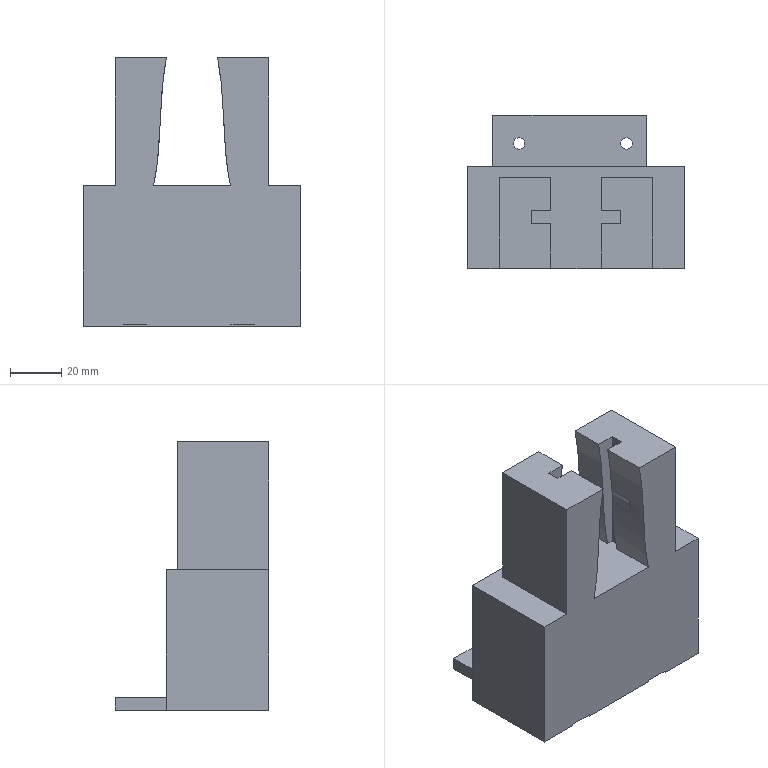Component | SolidWorks | ReagentBottleClampBlock-1 | 1 solid | 60 faces | box 85 x 60 x 105 mm | volume 252252 mm3 | plane 51 | cylinder 5 | spline 4 | commonest cylinder face diameters 4.5 x4 22.6 x1
build123d program:
from build123d import *

# Parameters (mm, degrees)
SKETCH1_2_W             = 60
SKETCH1_2_H             = 40
BOSS_EXTRUDE1_DEPTH     = 50
SKETCH3_W               = 35
SKETCH3_H               = 5
CUT_EXTRUDE1_2_DEPTH    = 50
CUT_EXTRUDE2_2_DEPTH    = 50
SKETCH6_W               = 85
SKETCH6_H               = 40
BOSS_EXTRUDE2_DEPTH     = 55
SKETCH7_W               = 60
SKETCH7_H               = 4.5
CUT_EXTRUDE3_DEPTH      = 50
SKETCH8_W               = 60
SKETCH8_H               = 5
BOSS_EXTRUDE3_DEPTH     = 20
SKETCH9_R               = 2.25
CUT_EXTRUDE4_DEPTH      = 20
SKETCH1_W               = 9
SKETCH1_H               = 14
SKETCH1_H_2             = 14.5
SKETCH1_H_3             = 5
CUT_EXTRUDE1_DEPTH      = 0.6
CUT_EXTRUDE2_DEPTH      = 5
CUT_EXTRUDE2_DEPTH_BACK = 5
SKETCH2_R               = 11.3


with BuildPart() as part:
    # Sketch1_2 → Boss-Extrude1 (new body)
    with BuildSketch(Plane.XY):
        Rectangle(SKETCH1_2_W, SKETCH1_2_H)
    extrude(amount=BOSS_EXTRUDE1_DEPTH)

    # Sketch3 → Cut-Extrude1_2 (cut)
    with BuildSketch(Plane.XY.offset(50)):
        Rectangle(SKETCH3_W, SKETCH3_H)
    extrude(amount=-CUT_EXTRUDE1_2_DEPTH, mode=Mode.SUBTRACT)

    # Sketch4 → Cut-Extrude2_2 (cut)
    with BuildSketch(Plane(origin=(0, 20, 0), x_dir=(1, 0, 0), z_dir=(0, 1, 0))):
        with BuildLine():
            Line((-10, 0), (10, 0))
            add(Edge.make_bspline(
                [(10, 0), (13.3, -16.524), (11.518, -33.504), (15, -50)],
                knots=[0, 0, 0, 0, 1, 1, 1, 1], degree=3))
            Line((15, -50), (-15, -50))
            add(Edge.make_bspline(
                [(-10, 0), (-13.3, -16.524), (-11.518, -33.504), (-15, -50)],
                knots=[0, 0, 0, 0, 1, 1, 1, 1], degree=3))
        make_face()
    extrude(amount=-CUT_EXTRUDE2_2_DEPTH, mode=Mode.SUBTRACT)


with BuildPart() as cut_extrude2_2_piece_1:
    # of the separate pieces the step leaves, piece 1, a body of its own (cut_extrude2_2_pieces)
    add(part.part.solids().sort_by_distance((-30, -20, 0))[0])



with BuildPart() as cut_extrude2_2_piece_2:
    # of the separate pieces the step leaves, piece 2, a body of its own (cut_extrude2_2_pieces)
    add(part.part.solids().sort_by_distance((10, -20, 0))[0])


with BuildPart() as cut_extrude2_2_piece_1_1:
    add(cut_extrude2_2_piece_1.part)

    add(cut_extrude2_2_piece_2.part)  # Boss-Extrude2 merges Cut-Extrude2_2 piece 2
    # Sketch6 → Boss-Extrude2 (add)
    with BuildSketch(Plane.XY.offset(50)):
        Rectangle(SKETCH6_W, SKETCH6_H)
    extrude(amount=BOSS_EXTRUDE2_DEPTH)

    # Sketch7 → Cut-Extrude3 (cut)
    with BuildSketch(Plane(origin=(0, 0, 0), x_dir=(-1, 0, 0), z_dir=(0, 0, -1))):
        with Locations((0, 17.75)):
            Rectangle(SKETCH7_W, SKETCH7_H)
    extrude(amount=-CUT_EXTRUDE3_DEPTH, mode=Mode.SUBTRACT)

    # Sketch8 → Boss-Extrude3 (add)
    with BuildSketch(Plane(origin=(0, 20, 0), x_dir=(1, 0, 0), z_dir=(0, 1, 0))):
        with Locations((2.5, -102.5)):
            Rectangle(SKETCH8_W, SKETCH8_H)
    extrude(amount=BOSS_EXTRUDE3_DEPTH)

    # Sketch9 → Cut-Extrude4 (cut)
    with BuildSketch(Plane(origin=(0, 0, 100), x_dir=(-1, 0, 0), z_dir=(0, 0, -1))):
        with Locations((-22.25, 29)):
            Circle(SKETCH9_R)
        with Locations((19.75, 29)):
            Circle(SKETCH9_R)
    extrude(amount=-CUT_EXTRUDE4_DEPTH, mode=Mode.SUBTRACT)

    # Sketch1 → Cut-Extrude1 (cut)
    with BuildSketch(Plane.XY.offset(105)):
        with Locations((22.25, 3)):
            Rectangle(SKETCH1_W, SKETCH1_H)
        with Locations((22.25, 28.75)):
            Rectangle(SKETCH1_W, SKETCH1_H_2)
        with Locations((22.25, -18)):
            Rectangle(SKETCH1_W, SKETCH1_H_3)
        with Locations((-19.75, 3)):
            Rectangle(SKETCH1_W, SKETCH1_H)
        with Locations((-19.75, 28.75)):
            Rectangle(SKETCH1_W, SKETCH1_H_2)
        with Locations((-19.75, -18)):
            Rectangle(SKETCH1_W, SKETCH1_H_3)
    extrude(amount=-CUT_EXTRUDE1_DEPTH, mode=Mode.SUBTRACT)

    # Sketch2 → Cut-Extrude2 (cut, two sides: drawn at the far end of the back side and taken through both)
    with BuildSketch(Plane(origin=(0, -7.5, 0), x_dir=(1, 0, 0), z_dir=(0, 1, 0)).offset(-CUT_EXTRUDE2_DEPTH_BACK)):
        with Locations((-1.5, -23.984)):
            Circle(SKETCH2_R)
    extrude(amount=CUT_EXTRUDE2_DEPTH + CUT_EXTRUDE2_DEPTH_BACK, mode=Mode.SUBTRACT)


solid = cut_extrude2_2_piece_1_1.part

# Placed as in the assembly
solid = solid.moved(Location((362.347, 1094.769, -2074.834), (-180, 0, 180)))